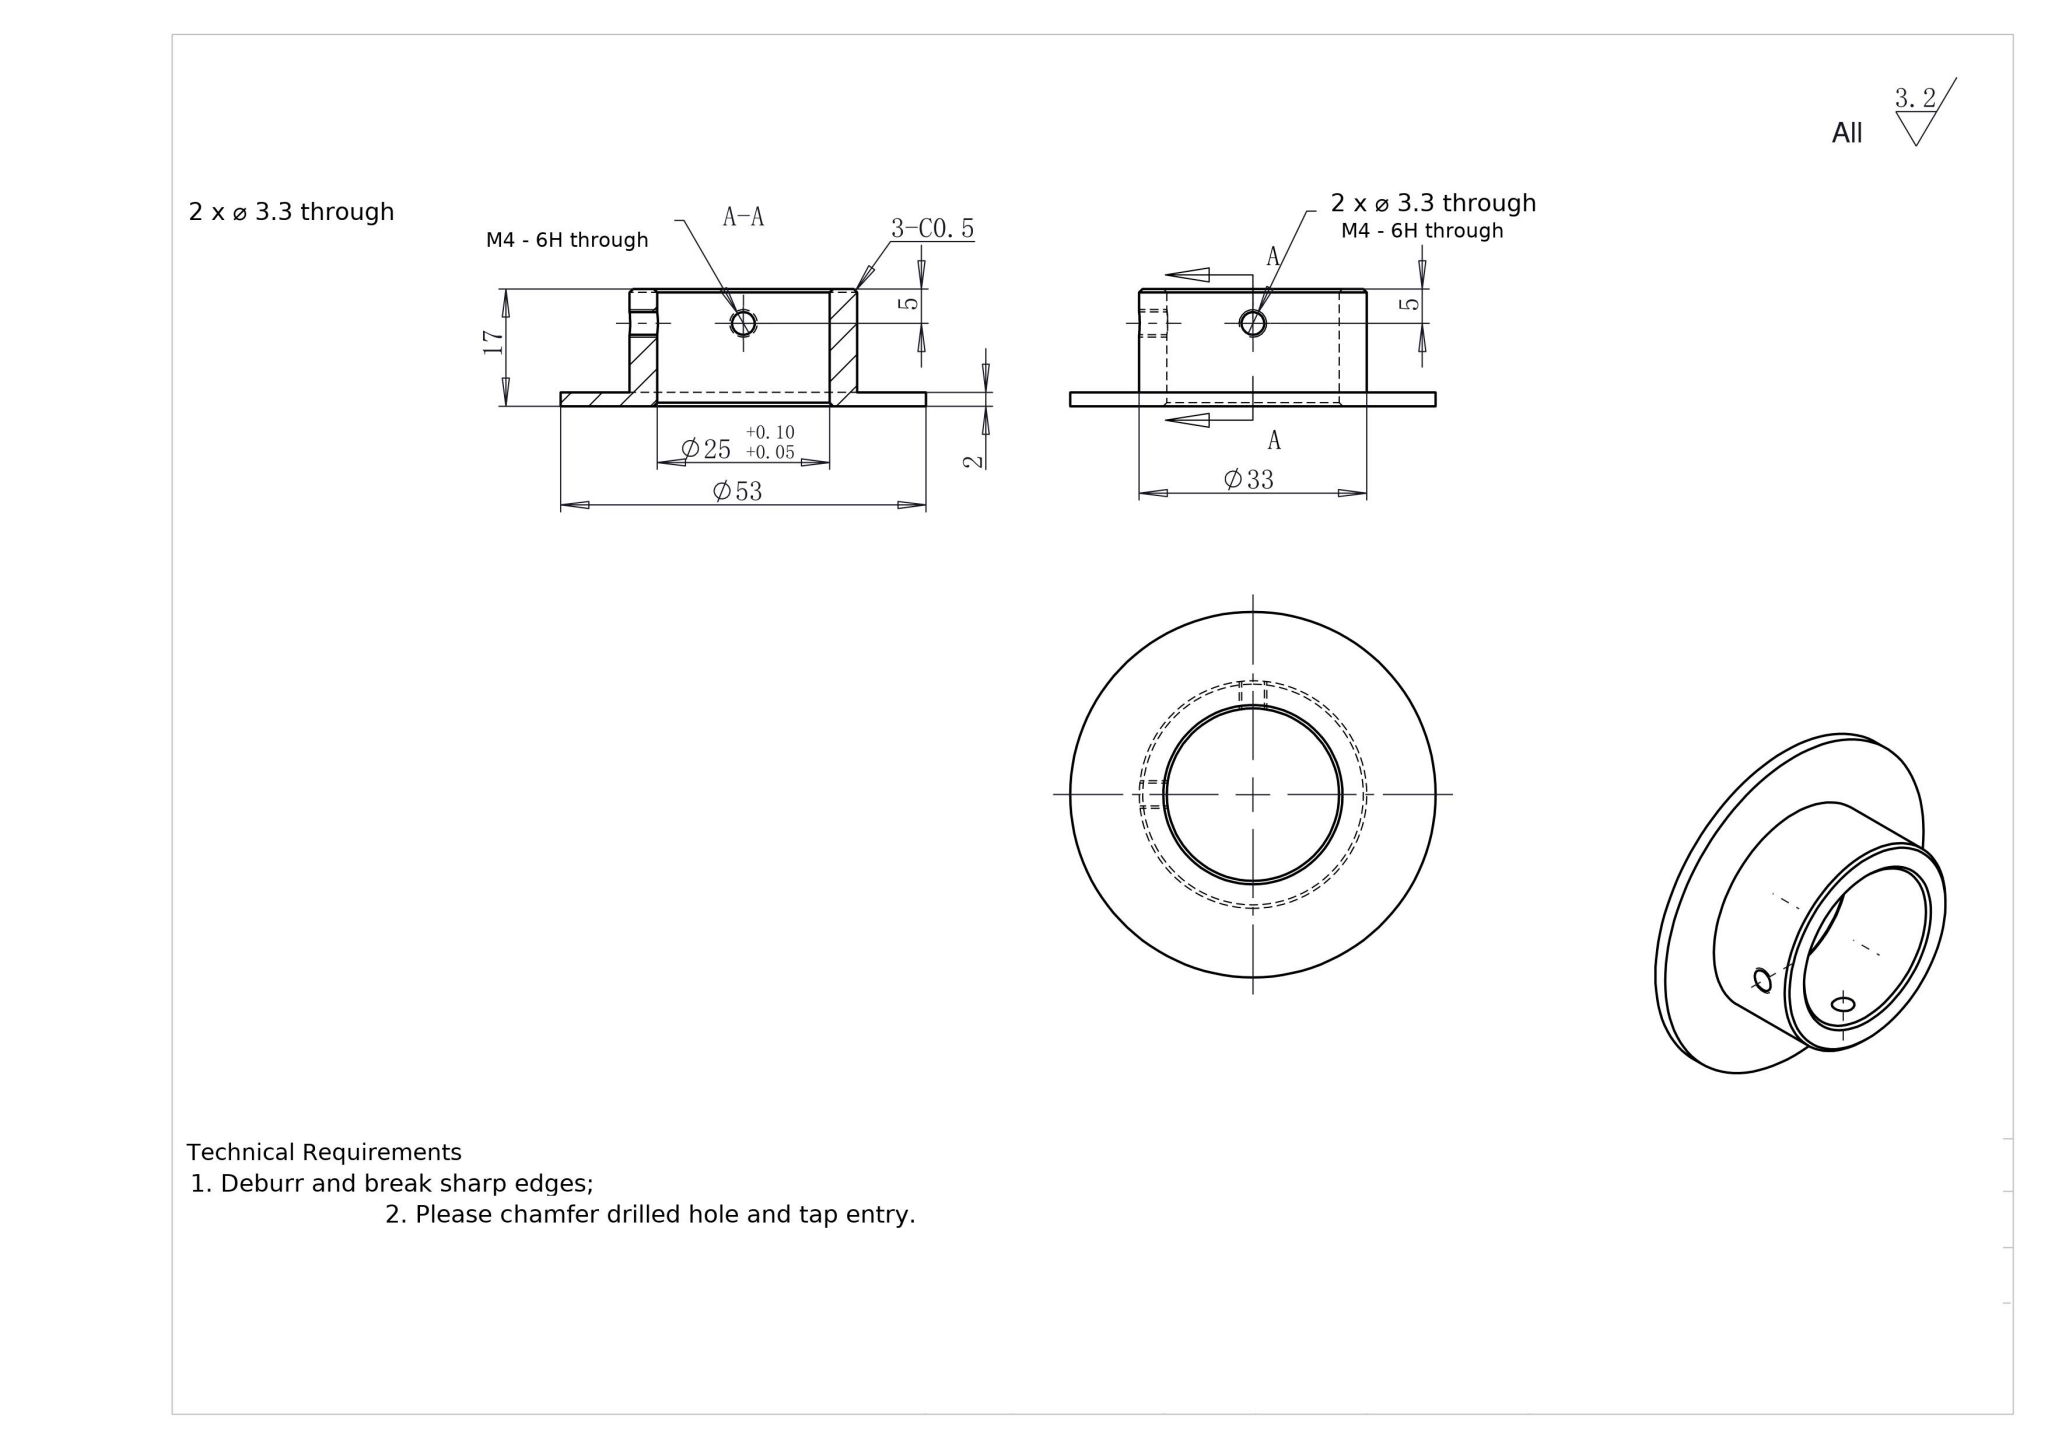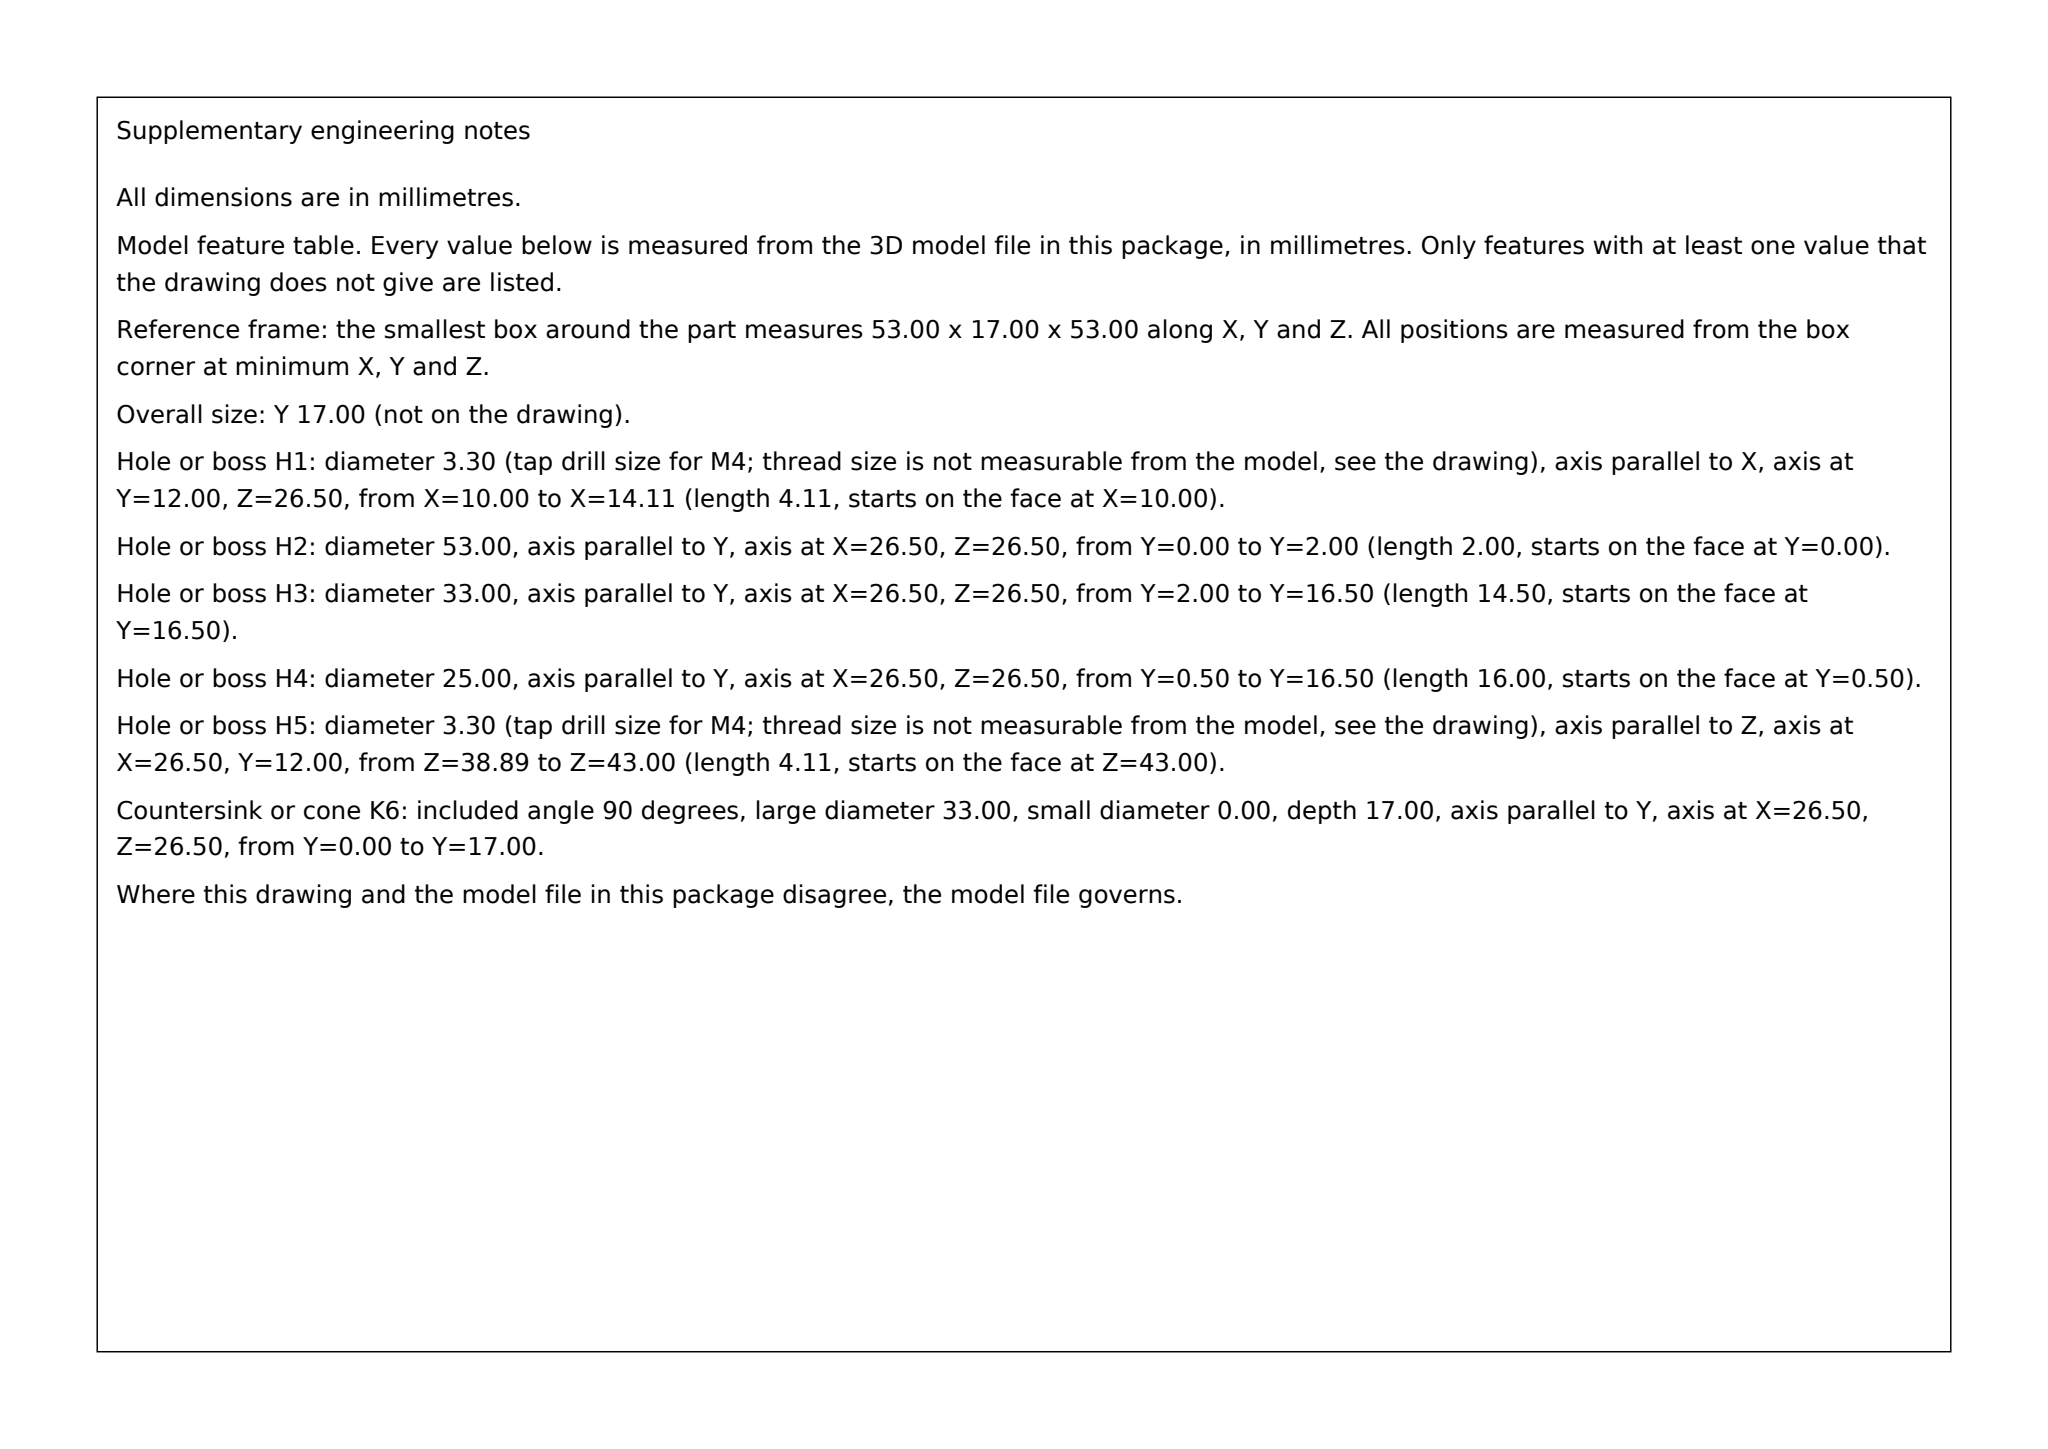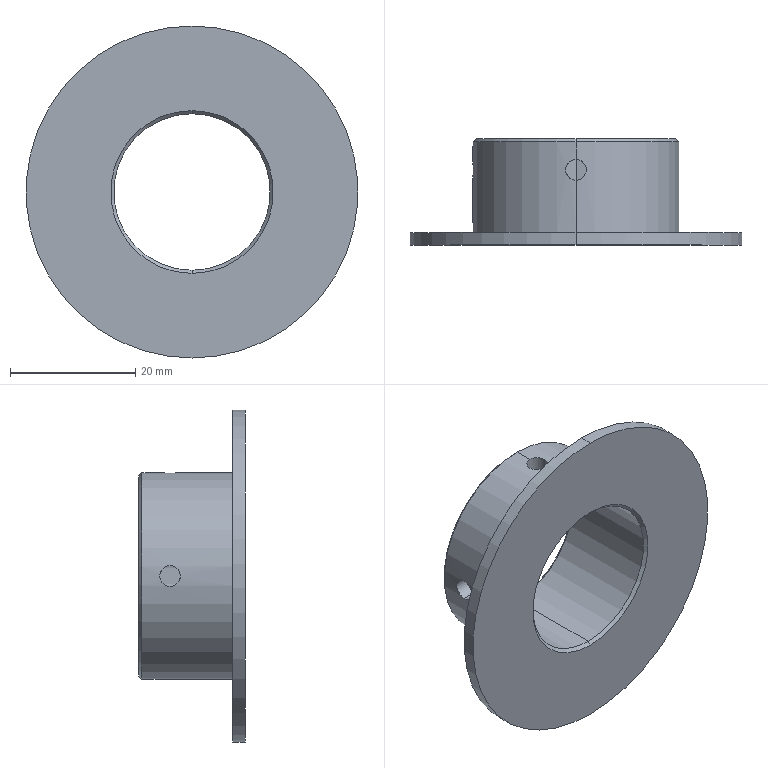Part | SolidWorks | mm | 1 solid | 19 faces | box 53 x 17 x 53 mm | volume 8796 mm3 | cylinder 10 | cone 6 | plane 3 | commonest cylinder face diameters 3.3 x4 53 x2 33 x2 25 x2
build123d program:
from build123d import *

# Parameters (mm, degrees)
M4_TAPPED_HOLE1_REACH  = 58.156
M4_TAPPED_HOLE1_BORE_R = 1.65
CIRPATTERN1_COUNT      = 2
CIRPATTERN1_ANGLE      = 90
CHAMFER1_SIZE          = 0.5


with BuildPart() as part:
    # Sketch1 → Revolve1 (revolve)
    with BuildSketch(Plane.XY, mode=Mode.PRIVATE) as revolve1_sk:
        Polygon((26.5, 0), (12.5, 0), (12.5, 17), (16.5, 17), (16.5, 2), (26.5, 2), align=None)
    revolve(revolve1_sk.sketch.rotate(Axis((0, 0, 0), (0, 1, 0)), 90), axis=Axis((0, 0, 0), (0, 1, 0)))

    # M4 Tapped Hole1 bore → M4 Tapped Hole1 (cut, up to next)
    with BuildSketch(Plane.XY.offset(20), mode=Mode.PRIVATE) as m4_tapped_hole1_sk1:
        with Locations((0, 12)):
            Circle(M4_TAPPED_HOLE1_BORE_R)
    m4_tapped_hole1_tool1 = extrude(m4_tapped_hole1_sk1.sketch, amount=-M4_TAPPED_HOLE1_REACH, mode=Mode.PRIVATE) & part.part
    m4_tapped_hole1 = m4_tapped_hole1_tool1.solids().sort_by_distance((0, 12, 20))[0]
    add(m4_tapped_hole1, mode=Mode.SUBTRACT)

    # CirPattern1: M4 Tapped Hole1 ×2 about axis
    cirpattern1_axis = Axis((0, 0, 0), (0, -1, 0))
    for i in range(1, CIRPATTERN1_COUNT):
        add(m4_tapped_hole1.rotate(cirpattern1_axis, i * CIRPATTERN1_ANGLE / (CIRPATTERN1_COUNT - 1)), mode=Mode.SUBTRACT)

    # Chamfer1
    chamfer1_edges = [part.edges().sort_by_distance(p)[0] for p in [
        (0, 0, 12.5),
        (0, 17, 16.5),
        (0, 17, 12.5),
    ]]
    chamfer(chamfer1_edges, length=CHAMFER1_SIZE)


solid = part.part